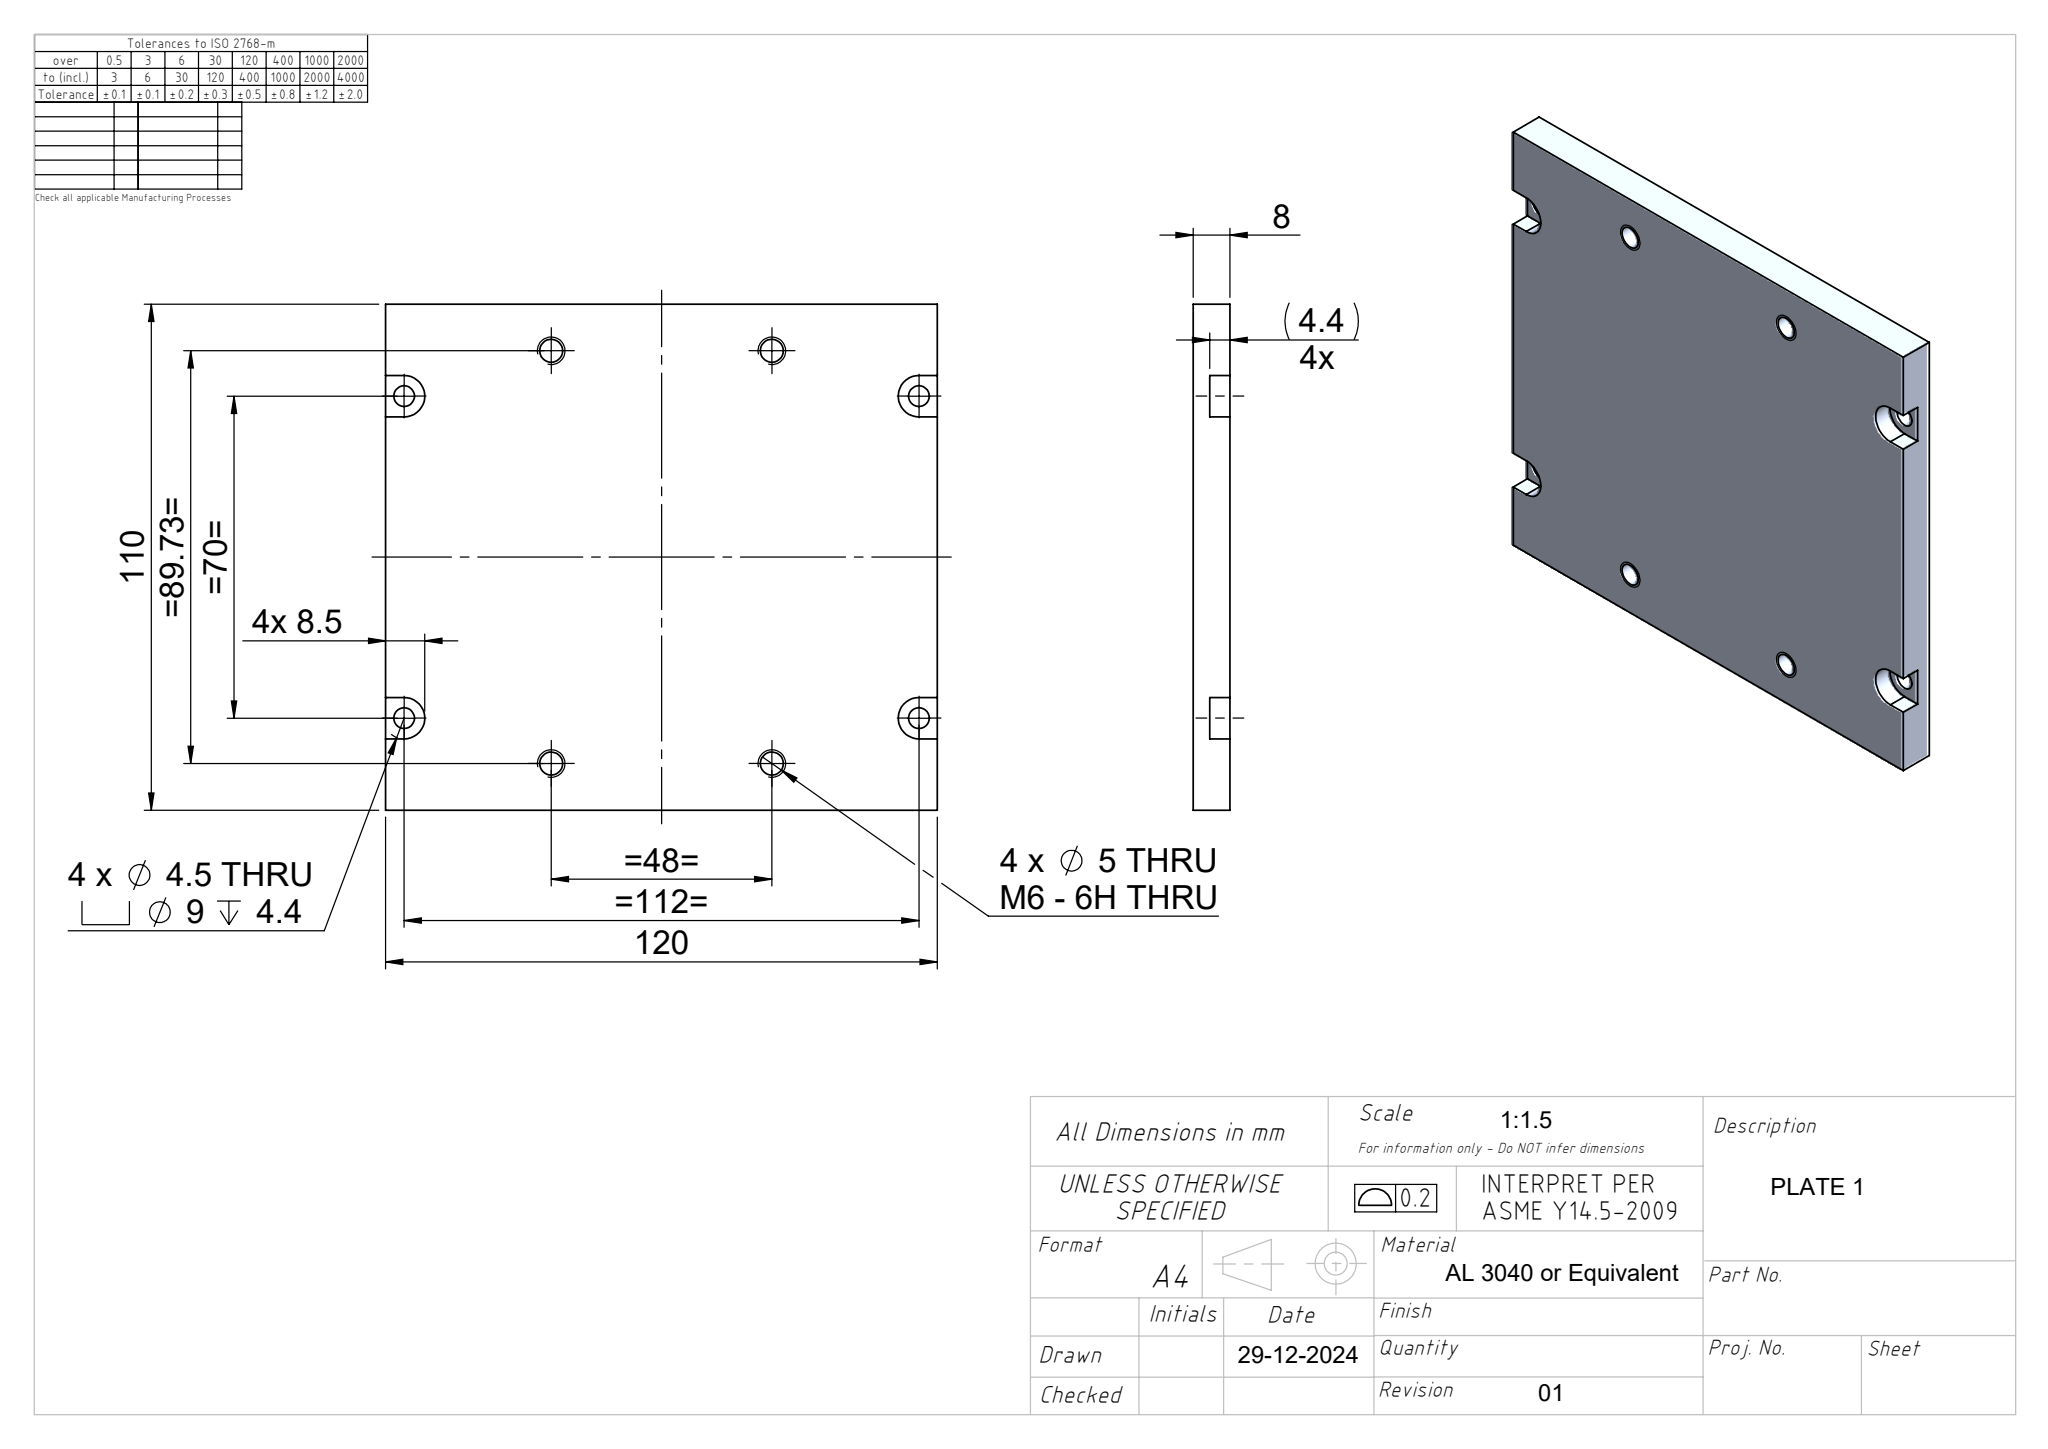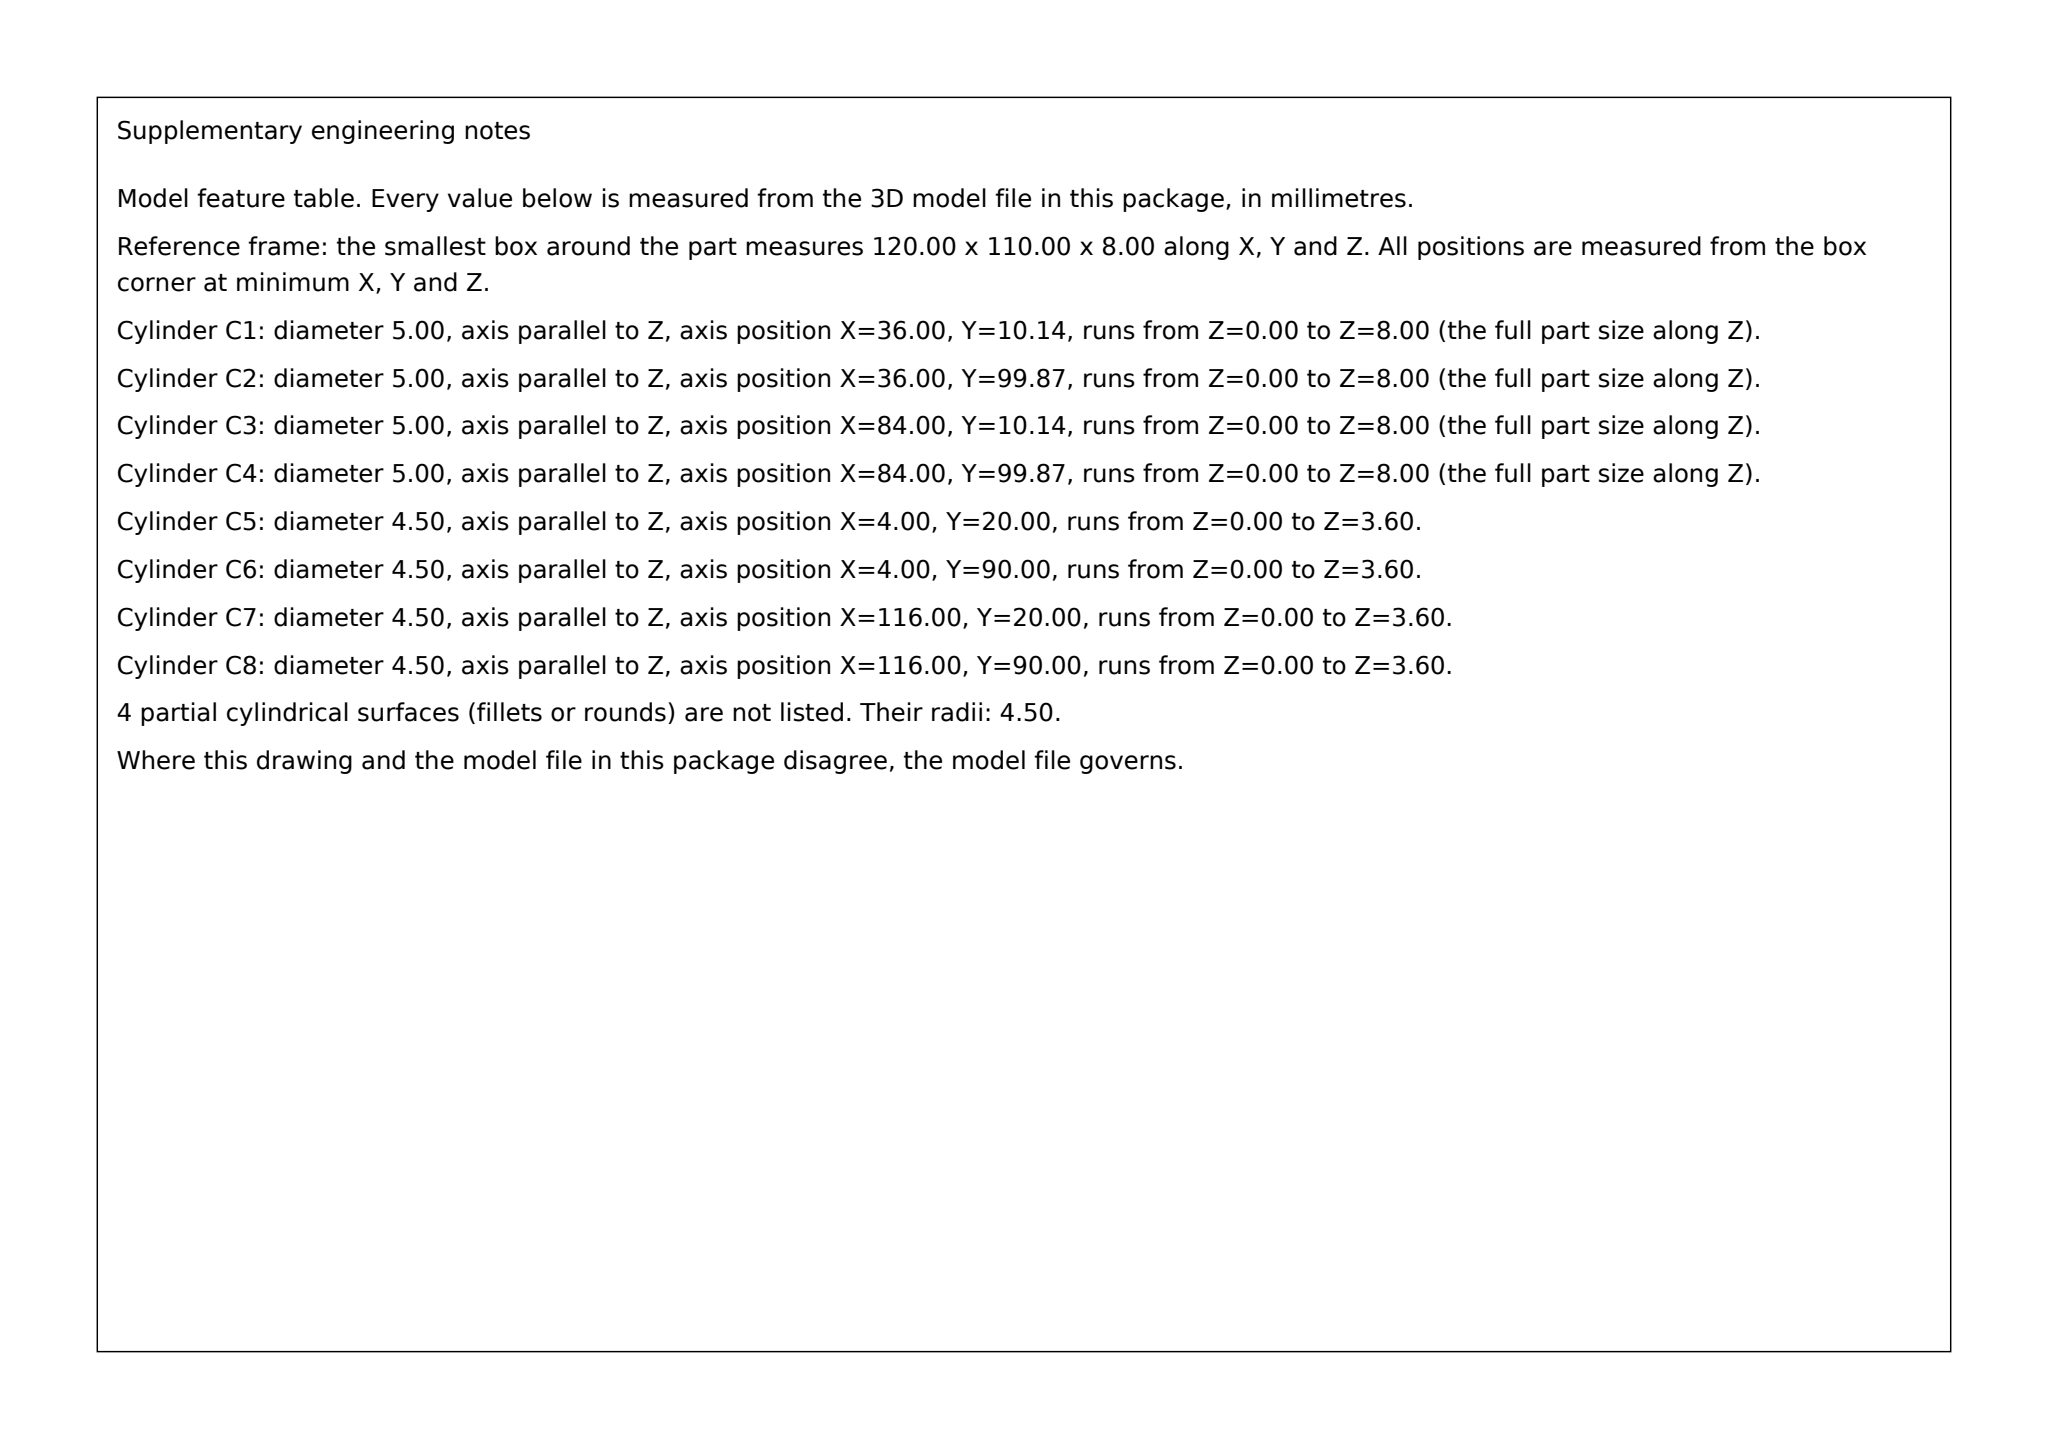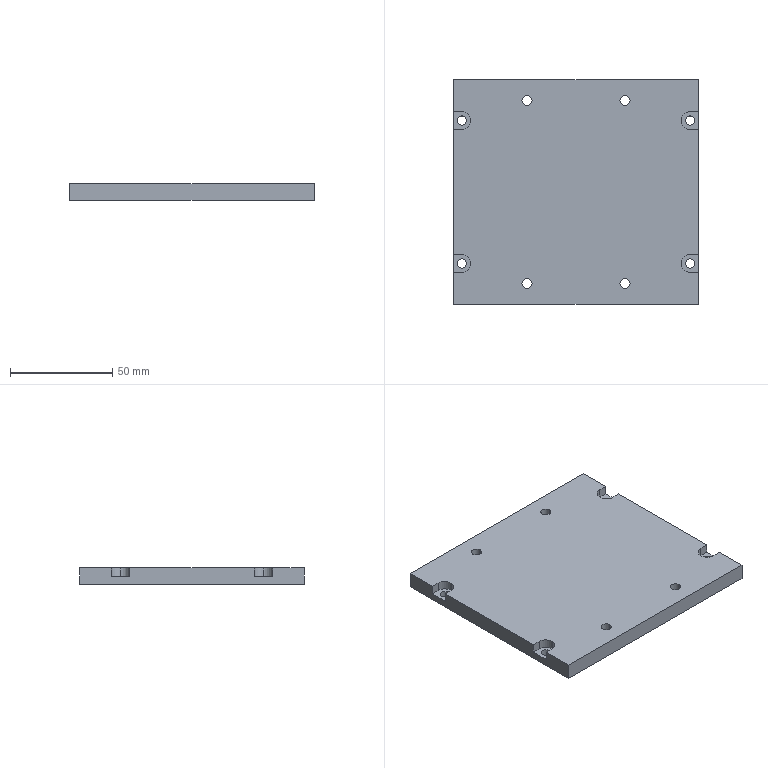Part | SolidWorks | mm | 1 solid | 40 faces | box 120 x 110 x 8 mm | volume 103549 mm3 | cylinder 22 | plane 18 | commonest cylinder face diameters 5 x8 4.5 x8 9 x6
build123d program:
from build123d import *

# Parameters (mm, degrees)
SKETCH1_W                                           = 120
SKETCH1_H                                           = 110
BOSS_EXTRUDE1_DEPTH                                 = 8
CBORE_FOR_M4_HEX_SOCKET_HEAD_CAP_SCREW1_D           = 4.5
CBORE_FOR_M4_HEX_SOCKET_HEAD_CAP_SCREW1_CBORE_D     = 9
CBORE_FOR_M4_HEX_SOCKET_HEAD_CAP_SCREW1_CBORE_DEPTH = 4.4
SKETCH4_W                                           = 4
SKETCH4_H                                           = 9
CUT_EXTRUDE1_DEPTH                                  = 4.4
M6_TAPPED_HOLE1_D                                   = 5


with BuildPart() as part:
    # Sketch1 → Boss-Extrude1 (new body)
    with BuildSketch(Plane.XY):
        with Locations((0, 55)):
            Rectangle(SKETCH1_W, SKETCH1_H)
    extrude(amount=BOSS_EXTRUDE1_DEPTH)

    # CBORE for M4 Hex Socket Head Cap Screw1 (through all)
    with Locations(Plane.XY.offset(8)):
        with Locations((-56, 90), (-56, 20), (56, 90), (56, 20)):
            CounterBoreHole(CBORE_FOR_M4_HEX_SOCKET_HEAD_CAP_SCREW1_D / 2, CBORE_FOR_M4_HEX_SOCKET_HEAD_CAP_SCREW1_CBORE_D / 2, CBORE_FOR_M4_HEX_SOCKET_HEAD_CAP_SCREW1_CBORE_DEPTH)

    # Sketch4 → Cut-Extrude1 (cut)
    with BuildSketch(Plane.XY.offset(8)):
        with Locations((58, 90)):
            Rectangle(SKETCH4_W, SKETCH4_H)
        with Locations((58, 20)):
            Rectangle(SKETCH4_W, SKETCH4_H)
        with Locations((-58, 20)):
            Rectangle(SKETCH4_W, SKETCH4_H)
        with Locations((-58, 90)):
            Rectangle(SKETCH4_W, SKETCH4_H)
    extrude(amount=-CUT_EXTRUDE1_DEPTH, mode=Mode.SUBTRACT)

    # M6 Tapped Hole1 (through all)
    with Locations(Plane.XY.offset(8)):
        with Locations((-24, 10.135), (24, 10.135), (24, 99.865), (-24, 99.865)):
            Hole(M6_TAPPED_HOLE1_D / 2)


solid = part.part